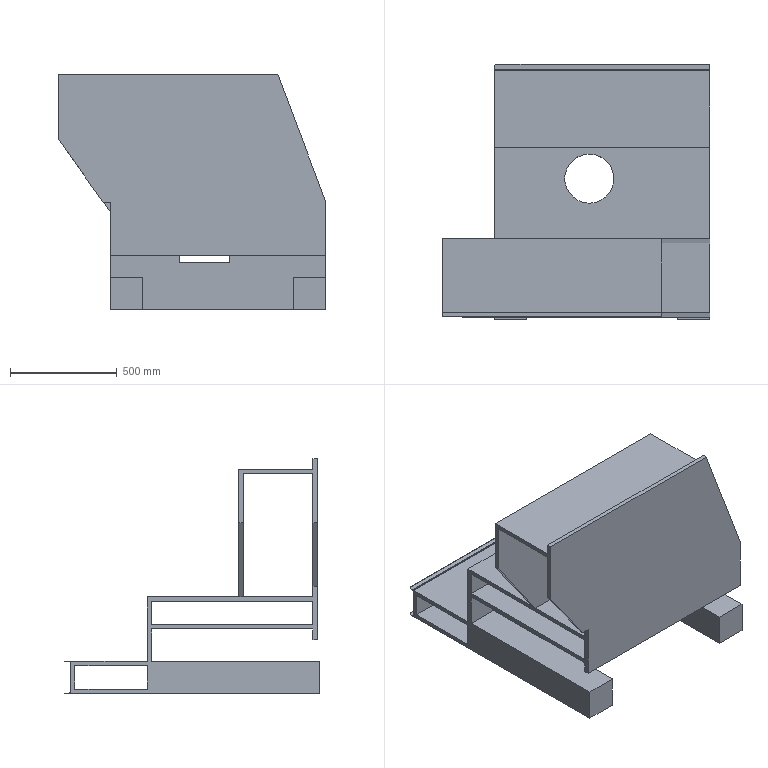Component | SolidWorks | Seat-1 | 2 solids | 67 faces | box 1255 x 1197 x 1100 mm | volume 125403476 mm3 | plane 55 | cylinder 12 | commonest cylinder face diameters 20 x4 230 x4 6 x2 12 x2 | material 45
build123d program:
from build123d import *

# Parameters (mm, degrees)
SKETCH1_W           = 110
SKETCH1_H           = 340
SKETCH1_H_2         = 755
BOSS_EXTRUDE1_DEPTH = 1008
SKETCH2_R           = 115
CUT_EXTRUDE1_DEPTH  = 1563.464
SKETCH3_W           = 1008
SKETCH3_H           = 20
BOSS_EXTRUDE2_DEPTH = 50
BOSS_EXTRUDE3_DEPTH = 1030
BOSS_EXTRUDE4_DEPTH = 20
BOSS_EXTRUDE5_DEPTH = 20
FILLET1_R           = 20
BOSS_EXTRUDE6_DEPTH = 1008
FILLET2_R           = 10
CUT_EXTRUDE2_DEPTH  = 1609.629
SKETCH10_W          = 80
SKETCH10_H          = 238
CUT_EXTRUDE3_DEPTH  = 20
SKETCH11_W          = 272
SKETCH11_H          = 418
CUT_EXTRUDE4_DEPTH  = 20
SKETCH12_W          = 150
SKETCH12_H          = 150
BOSS_EXTRUDE7_DEPTH = 787


with BuildPart() as part:
    # Sketch1 → Boss-Extrude1 (new body)
    with BuildSketch(Plane.XY):
        Polygon((0, 0), (150, 0), (150, -380), (-152, -380), (-152, -1155), (-302, -1155), (-302, -360), (0, -360), align=None)
        with Locations((75, -190)):
            Rectangle(SKETCH1_W, SKETCH1_H, mode=Mode.SUBTRACT)
        with Locations((-227, -757.5)):
            Rectangle(SKETCH1_W, SKETCH1_H_2, mode=Mode.SUBTRACT)
    extrude(amount=BOSS_EXTRUDE1_DEPTH)

    # Sketch2 → Cut-Extrude1 (cut, through all)
    with BuildSketch(Plane.ZY.offset(152)):
        with Locations((443, -507)):
            Circle(SKETCH2_R)
    extrude(amount=CUT_EXTRUDE1_DEPTH, mode=Mode.SUBTRACT)

    # Sketch3 → Boss-Extrude2 (add)
    with BuildSketch(Plane.ZY.offset(152)):
        with Locations((504, -1145)):
            Rectangle(SKETCH3_W, SKETCH3_H)
    boss_extrude2 = extrude(amount=-BOSS_EXTRUDE2_DEPTH)

    # Mirror1: Boss-Extrude2 across plane
    add(boss_extrude2.mirror(Plane(origin=(-227, 0, 0), x_dir=(0, 0, 1), z_dir=(1, 0, 0))))

    # Sketch4 → Boss-Extrude3 (add)
    with BuildSketch(Plane(origin=(0, 0, -247), x_dir=(-1, 0, 0), z_dir=(0, 0, -1))):
        Polygon((302, -788), (900, -788), (900, -1135), (950, -1135), (950, -1155), (352, -1155), (352, -1135), (880, -1135), (880, -808), (302, -808), align=None)
    extrude(amount=-BOSS_EXTRUDE3_DEPTH)

    # Sketch5 → Boss-Extrude4 (add)
    with BuildSketch(Plane(origin=(0, -1135, 0), x_dir=(1, 0, 0), z_dir=(0, 1, 0))):
        Polygon((-950, -783), (-352, -1008), (-352, -783), align=None)
    extrude(amount=-BOSS_EXTRUDE4_DEPTH)

    # Sketch6 → Boss-Extrude5 (add)
    with BuildSketch(Plane(origin=(0, -788, 0), x_dir=(1, 0, 0), z_dir=(0, 1, 0))):
        Polygon((-900, -783), (-302, -783), (-302, -1008), align=None)
    extrude(amount=-BOSS_EXTRUDE5_DEPTH)

    # Fillet1
    fillet1_edges = [part.edges().sort_by_distance(p)[0] for p in [
        (-302, -798, -247),
        (-352, -1145, -247),
    ]]
    fillet(fillet1_edges, radius=FILLET1_R)

    # Sketch8 → Cut-Extrude2 (cut, through all)
    with BuildSketch(Plane(origin=(0, -788, 0), x_dir=(1, 0, 0), z_dir=(0, 1, 0))):
        Polygon((-302, 0), (-650, 247), (-302, 247), align=None)
    extrude(amount=-CUT_EXTRUDE2_DEPTH, mode=Mode.SUBTRACT)

    # Sketch10 → Cut-Extrude3 (cut)
    with BuildSketch(Plane.XZ.offset(380)):
        with Locations((-112, 439)):
            Rectangle(SKETCH10_W, SKETCH10_H)
    extrude(amount=-CUT_EXTRUDE3_DEPTH, mode=Mode.SUBTRACT)

    # Sketch11 → Cut-Extrude4 (cut)
    with BuildSketch(Plane(origin=(0, -788, 0), x_dir=(1, 0, 0), z_dir=(0, 1, 0))):
        with Locations((-438, -449)):
            Rectangle(SKETCH11_W, SKETCH11_H)
    extrude(amount=-CUT_EXTRUDE4_DEPTH, mode=Mode.SUBTRACT)

    # Sketch12 → Boss-Extrude7 (add)
    with BuildSketch(Plane.XZ.offset(380)):
        with Locations((75, 75)):
            Rectangle(SKETCH12_W, SKETCH12_H)
        with Locations((75, 933)):
            Rectangle(SKETCH12_W, SKETCH12_H)
    extrude(amount=BOSS_EXTRUDE7_DEPTH)


with BuildPart() as body_2:
    # Sketch7 → Boss-Extrude6 (new body)
    with BuildSketch(Plane(origin=(0, 0, 0), x_dir=(-1, 0, 0), z_dir=(0, 0, -1))):
        with BuildLine():
            Line((-150, 30), (-150, 6))
            ThreePointArc((-150, 6), (-148.243, 1.757), (-144, 0))
            Line((-144, 0), (-6, 0))
            ThreePointArc((-6, 0), (-1.757, 1.757), (0, 6))
            Line((0, 6), (0, 30))
            Line((0, 30), (-2, 30))
            Line((-2, 30), (-2, 5))
            ThreePointArc((-2, 5), (-2.879, 2.879), (-5, 2))
            Line((-5, 2), (-145, 2))
            ThreePointArc((-145, 2), (-147.121, 2.879), (-148, 5))
            Line((-148, 5), (-148, 30))
            Line((-148, 30), (-150, 30))
        make_face()
    extrude(amount=-BOSS_EXTRUDE6_DEPTH)

    # Fillet2
    fillet2_edges = [body_2.edges().sort_by_distance(p)[0] for p in [
        (1, 30, 0),
        (149, 30, 0),
        (1, 30, 1008),
        (149, 30, 1008),
    ]]
    fillet(fillet2_edges, radius=FILLET2_R)


solid = Compound([part.part, body_2.part])

# Placed as in the assembly
solid = solid.moved(Location((-533.813, 755.429, 450.267), (0, 90, 0)))